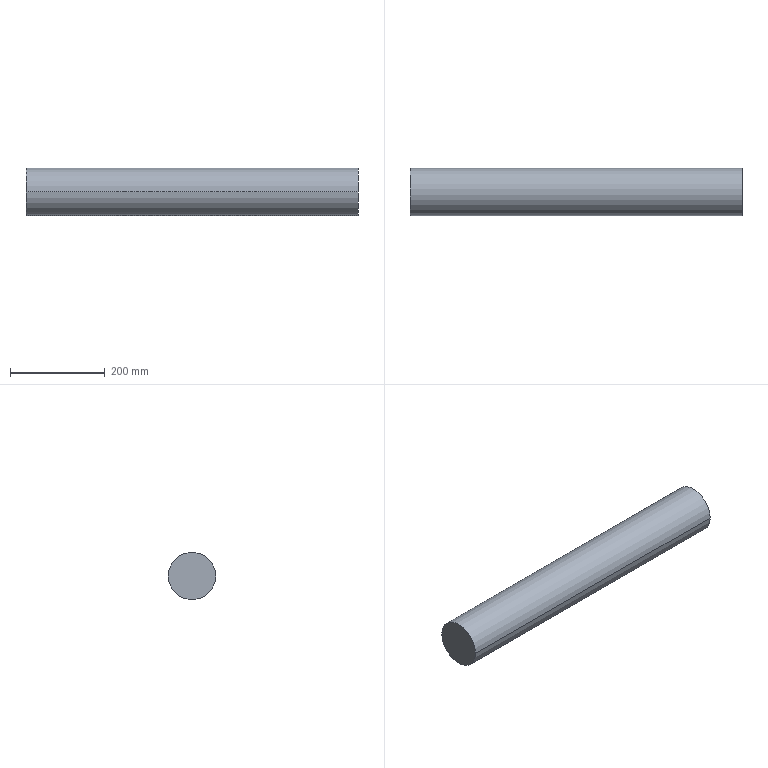Component | SolidWorks | CamAxis-1 | 1 solid | 4 faces | box 700 x 100 x 100 mm | volume 5497787 mm3 | cylinder 2 | plane 2 | commonest cylinder face diameters 100 x2
build123d program:
from build123d import *

# Parameters (mm, degrees)
SKETCH1_W = 50
SKETCH1_H = 700


with BuildPart() as part:
    # Sketch1 → Revolve1 (revolve)
    with BuildSketch(Plane.XZ, mode=Mode.PRIVATE) as revolve1_sk:
        with Locations((25, -300)):
            Rectangle(SKETCH1_W, SKETCH1_H)
    revolve(revolve1_sk.sketch.rotate(Axis((0, 0, 50), (0, 0, -1)), 180), axis=Axis((0, 0, 50), (0, 0, -1)))


solid = part.part

# Placed as in the assembly
solid = solid.moved(Location((-119.332, 870.769, 1116.347), (0, 90, 0)))
STEP:
#1=COLOUR_RGB('',0.7922,0.8196,0.9333);
#2=FILL_AREA_STYLE_COLOUR('',#1);
#3=FILL_AREA_STYLE('',(#2));
#4=SURFACE_STYLE_FILL_AREA(#3);
#5=SURFACE_SIDE_STYLE('',(#4));
#6=SURFACE_STYLE_USAGE(.BOTH.,#5);
#7=PRESENTATION_STYLE_ASSIGNMENT((#6));
#8=CARTESIAN_POINT('',(-2.73,32.314,43.951));
#9=VERTEX_POINT('',#8);
#10=CARTESIAN_POINT('',(-2.73,36.251,43.951));
#11=VERTEX_POINT('',#10);
#12=CARTESIAN_POINT('',(-2.73,34.282,43.951));
#13=DIRECTION('',(-1.,0.,0.));
#14=DIRECTION('',(0.,-1.,0.));
#15=AXIS2_PLACEMENT_3D('',#12,#13,#14);
#16=CIRCLE('',#15,1.969);
#17=EDGE_CURVE('',#9,#11,#16,.T.);
#18=ORIENTED_EDGE('',*,*,#17,.T.);
#19=CARTESIAN_POINT('',(-30.289,36.251,43.951));
#20=VERTEX_POINT('',#19);
#21=CARTESIAN_POINT('',(-2.73,36.251,43.951));
#22=DIRECTION('',(-1.,0.,0.));
#23=VECTOR('',#22,39.37);
#24=LINE('',#21,#23);
#25=EDGE_CURVE('',#11,#20,#24,.T.);
#26=ORIENTED_EDGE('',*,*,#25,.T.);
#27=CARTESIAN_POINT('',(-30.289,32.314,43.951));
#28=VERTEX_POINT('',#27);
#29=CARTESIAN_POINT('',(-30.289,34.282,43.951));
#30=DIRECTION('',(-1.,0.,0.));
#31=DIRECTION('',(0.,-1.,0.));
#32=AXIS2_PLACEMENT_3D('',#29,#30,#31);
#33=CIRCLE('',#32,1.969);
#34=EDGE_CURVE('',#28,#20,#33,.T.);
#35=ORIENTED_EDGE('',*,*,#34,.F.);
#36=CARTESIAN_POINT('',(-2.73,32.314,43.951));
#37=DIRECTION('',(-1.,0.,0.));
#38=VECTOR('',#37,39.37);
#39=LINE('',#36,#38);
#40=EDGE_CURVE('',#9,#28,#39,.T.);
#41=ORIENTED_EDGE('',*,*,#40,.F.);
#42=EDGE_LOOP('',(#18,#26,#35,#41));
#43=FACE_OUTER_BOUND('',#42,.T.);
#44=CARTESIAN_POINT('',(-2.73,34.282,43.951));
#45=DIRECTION('',(-1.,0.,0.));
#46=DIRECTION('',(0.,-1.,0.));
#47=AXIS2_PLACEMENT_3D('',#44,#45,#46);
#48=CYLINDRICAL_SURFACE('',#47,1.969);
#49=ADVANCED_FACE('',(#43),#48,.T.);
#50=ORIENTED_EDGE('',*,*,#25,.F.);
#51=CARTESIAN_POINT('',(-2.73,34.282,43.951));
#52=DIRECTION('',(-1.,0.,0.));
#53=DIRECTION('',(0.,-1.,0.));
#54=AXIS2_PLACEMENT_3D('',#51,#52,#53);
#55=CIRCLE('',#54,1.969);
#56=EDGE_CURVE('',#11,#9,#55,.T.);
#57=ORIENTED_EDGE('',*,*,#56,.T.);
#58=ORIENTED_EDGE('',*,*,#40,.T.);
#59=CARTESIAN_POINT('',(-30.289,34.282,43.951));
#60=DIRECTION('',(-1.,0.,0.));
#61=DIRECTION('',(0.,-1.,0.));
#62=AXIS2_PLACEMENT_3D('',#59,#60,#61);
#63=CIRCLE('',#62,1.969);
#64=EDGE_CURVE('',#20,#28,#63,.T.);
#65=ORIENTED_EDGE('',*,*,#64,.F.);
#66=EDGE_LOOP('',(#50,#57,#58,#65));
#67=FACE_OUTER_BOUND('',#66,.T.);
#68=CARTESIAN_POINT('',(-2.73,34.282,43.951));
#69=DIRECTION('',(-1.,0.,0.));
#70=DIRECTION('',(0.,-1.,0.));
#71=AXIS2_PLACEMENT_3D('',#68,#69,#70);
#72=CYLINDRICAL_SURFACE('',#71,1.969);
#73=ADVANCED_FACE('',(#67),#72,.T.);
#74=ORIENTED_EDGE('',*,*,#17,.F.);
#75=ORIENTED_EDGE('',*,*,#56,.F.);
#76=EDGE_LOOP('',(#74,#75));
#77=FACE_OUTER_BOUND('',#76,.T.);
#78=CARTESIAN_POINT('',(-2.73,36.251,43.951));
#79=DIRECTION('',(1.,0.,0.));
#80=DIRECTION('',(0.,1.,0.));
#81=AXIS2_PLACEMENT_3D('',#78,#79,#80);
#82=PLANE('',#81);
#83=ADVANCED_FACE('',(#77),#82,.T.);
#84=ORIENTED_EDGE('',*,*,#34,.T.);
#85=ORIENTED_EDGE('',*,*,#64,.T.);
#86=EDGE_LOOP('',(#84,#85));
#87=FACE_OUTER_BOUND('',#86,.T.);
#88=CARTESIAN_POINT('',(-30.289,34.282,43.951));
#89=DIRECTION('',(-1.,0.,0.));
#90=DIRECTION('',(0.,-1.,0.));
#91=AXIS2_PLACEMENT_3D('',#88,#89,#90);
#92=PLANE('',#91);
#93=ADVANCED_FACE('',(#87),#92,.T.);
#94=CLOSED_SHELL('',(#49,#73,#83,#93));
#95=MANIFOLD_SOLID_BREP('',#94);
#96=STYLED_ITEM('',(#7),#95);
#97=PRESENTATION_LAYER_ASSIGNMENT('','',(#96));
#98=(LENGTH_UNIT()NAMED_UNIT(*)SI_UNIT($,.METRE.));
#99=LENGTH_MEASURE_WITH_UNIT(LENGTH_MEASURE(0.0254),#98);
#100=DIMENSIONAL_EXPONENTS(1.,0.,0.,0.,0.,0.,0.);
#101=(CONVERSION_BASED_UNIT('',#99)LENGTH_UNIT()NAMED_UNIT(#100));
#102=UNCERTAINTY_MEASURE_WITH_UNIT(LENGTH_MEASURE(0.00001),#101,'','');
#103=(NAMED_UNIT(*)PLANE_ANGLE_UNIT()SI_UNIT($,.RADIAN.));
#104=(NAMED_UNIT(*)SI_UNIT($,.STERADIAN.)SOLID_ANGLE_UNIT());
#105=(GEOMETRIC_REPRESENTATION_CONTEXT(3)GLOBAL_UNCERTAINTY_ASSIGNED_CONTEXT((#102))GLOBAL_UNIT_ASSIGNED_CONTEXT((#101,#103,#104))REPRESENTATION_CONTEXT('',''));
#106=MECHANICAL_DESIGN_GEOMETRIC_PRESENTATION_REPRESENTATION('',(#96),#105);
#107=CARTESIAN_POINT('',(0.,0.,0.));
#108=DIRECTION('',(0.,0.,1.));
#109=DIRECTION('',(1.,0.,0.));
#110=AXIS2_PLACEMENT_3D('',#107,#108,#109);
#111=(LENGTH_UNIT()NAMED_UNIT(*)SI_UNIT($,.METRE.));
#112=LENGTH_MEASURE_WITH_UNIT(LENGTH_MEASURE(0.0254),#111);
#113=DIMENSIONAL_EXPONENTS(1.,0.,0.,0.,0.,0.,0.);
#114=(CONVERSION_BASED_UNIT('',#112)LENGTH_UNIT()NAMED_UNIT(#113));
#115=UNCERTAINTY_MEASURE_WITH_UNIT(LENGTH_MEASURE(0.00001),#114,'','');
#116=(NAMED_UNIT(*)PLANE_ANGLE_UNIT()SI_UNIT($,.RADIAN.));
#117=(NAMED_UNIT(*)SI_UNIT($,.STERADIAN.)SOLID_ANGLE_UNIT());
#118=(GEOMETRIC_REPRESENTATION_CONTEXT(3)GLOBAL_UNCERTAINTY_ASSIGNED_CONTEXT((#115))GLOBAL_UNIT_ASSIGNED_CONTEXT((#114,#116,#117))REPRESENTATION_CONTEXT('',''));
#119=ADVANCED_BREP_SHAPE_REPRESENTATION('',(#95,#110),#118);